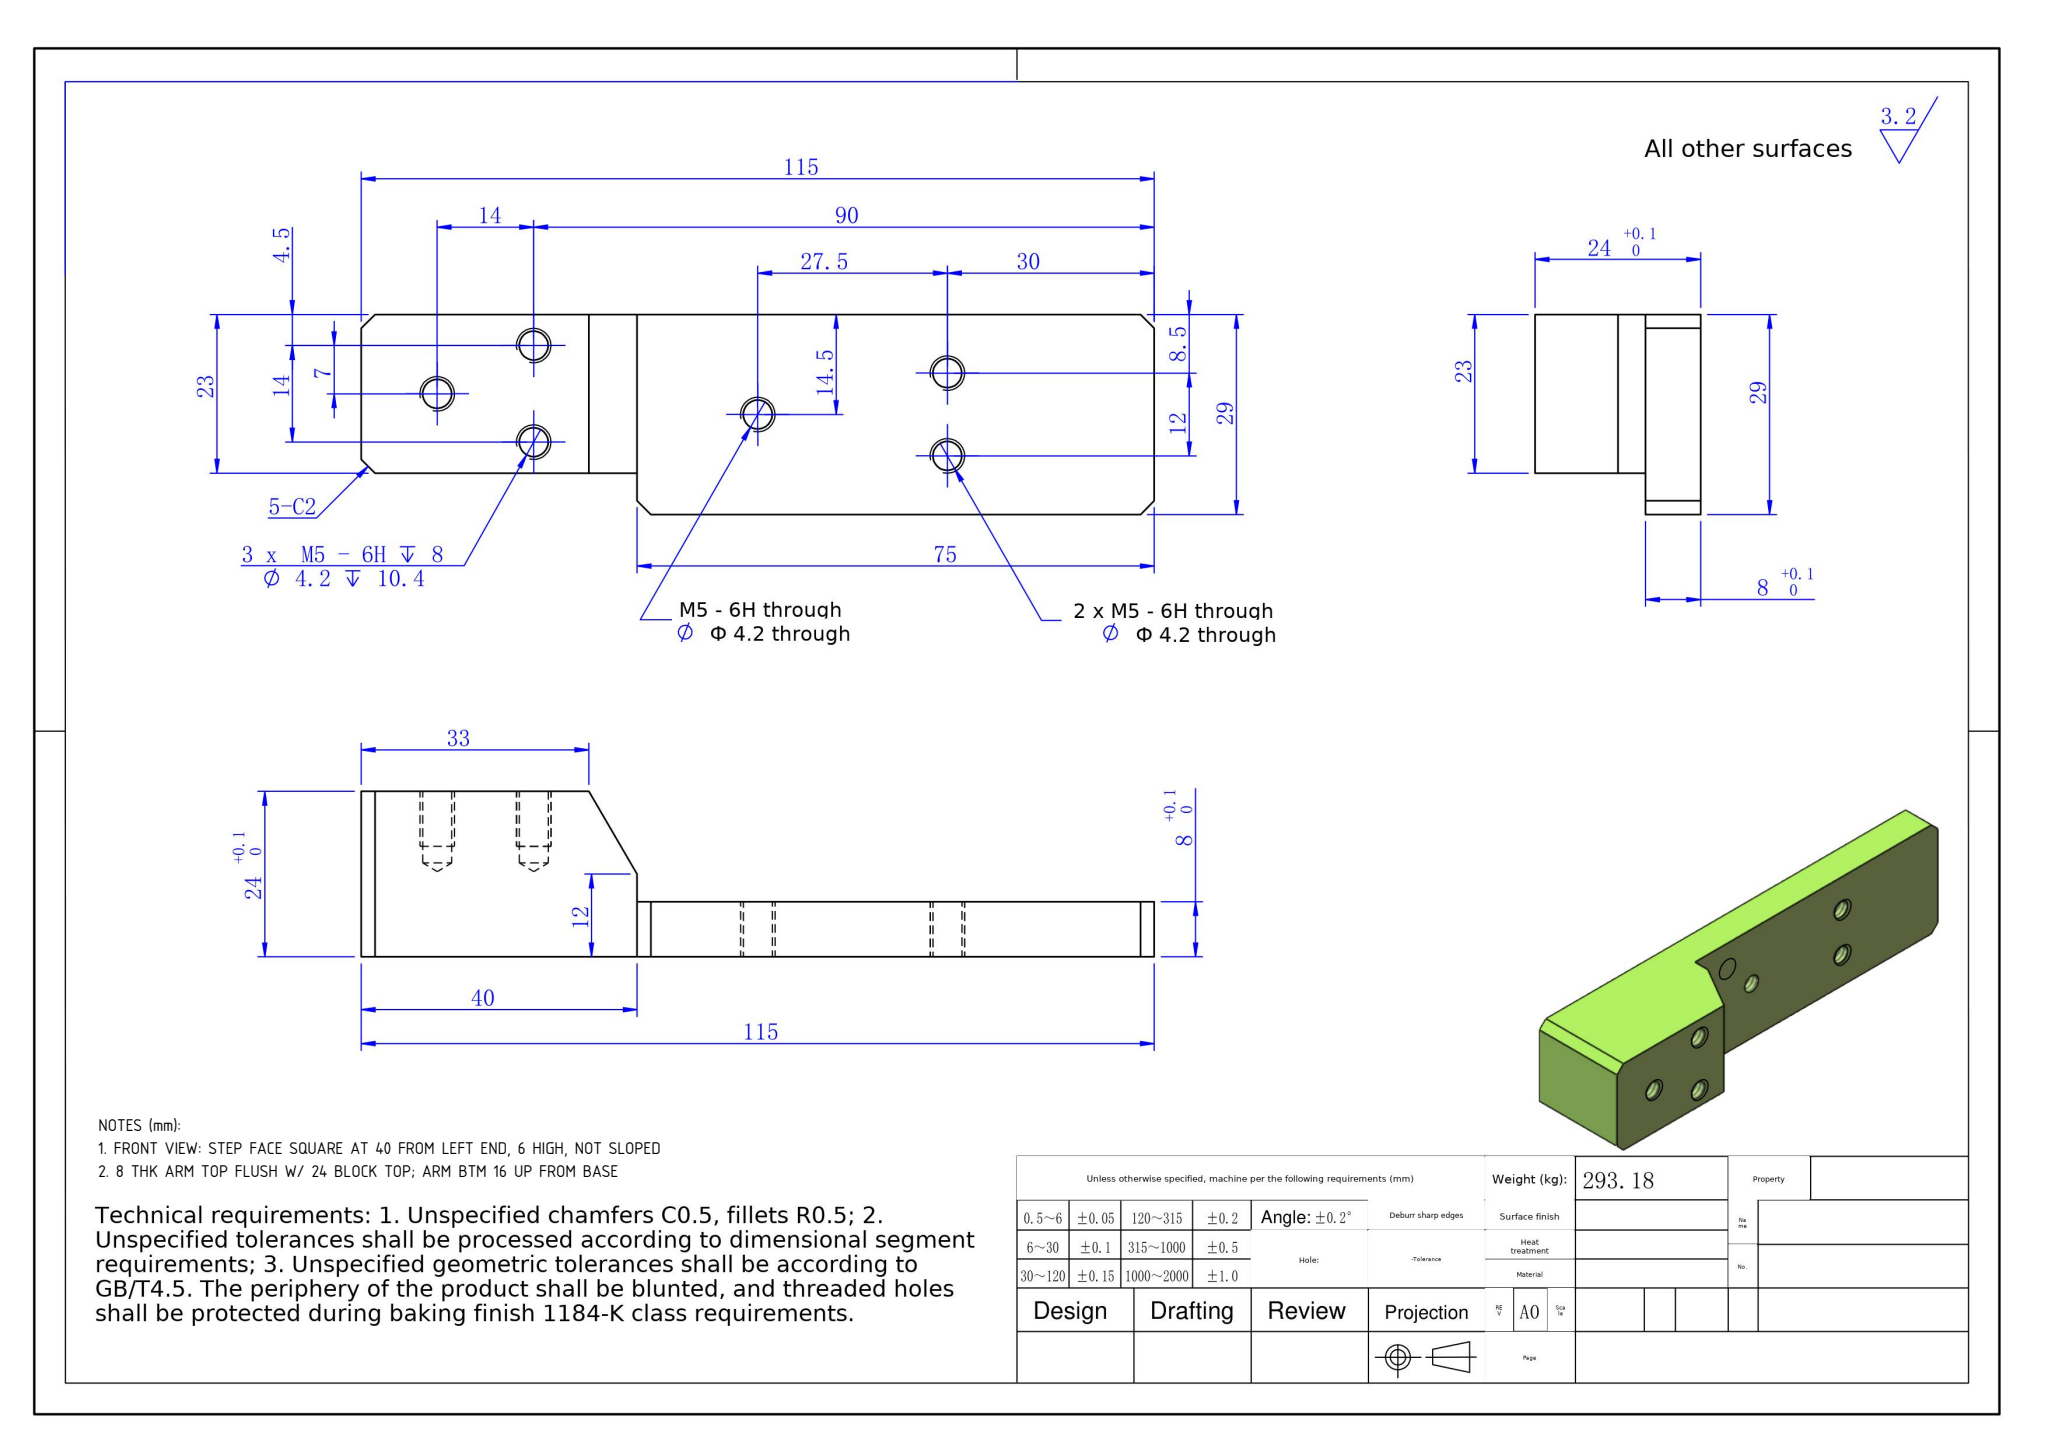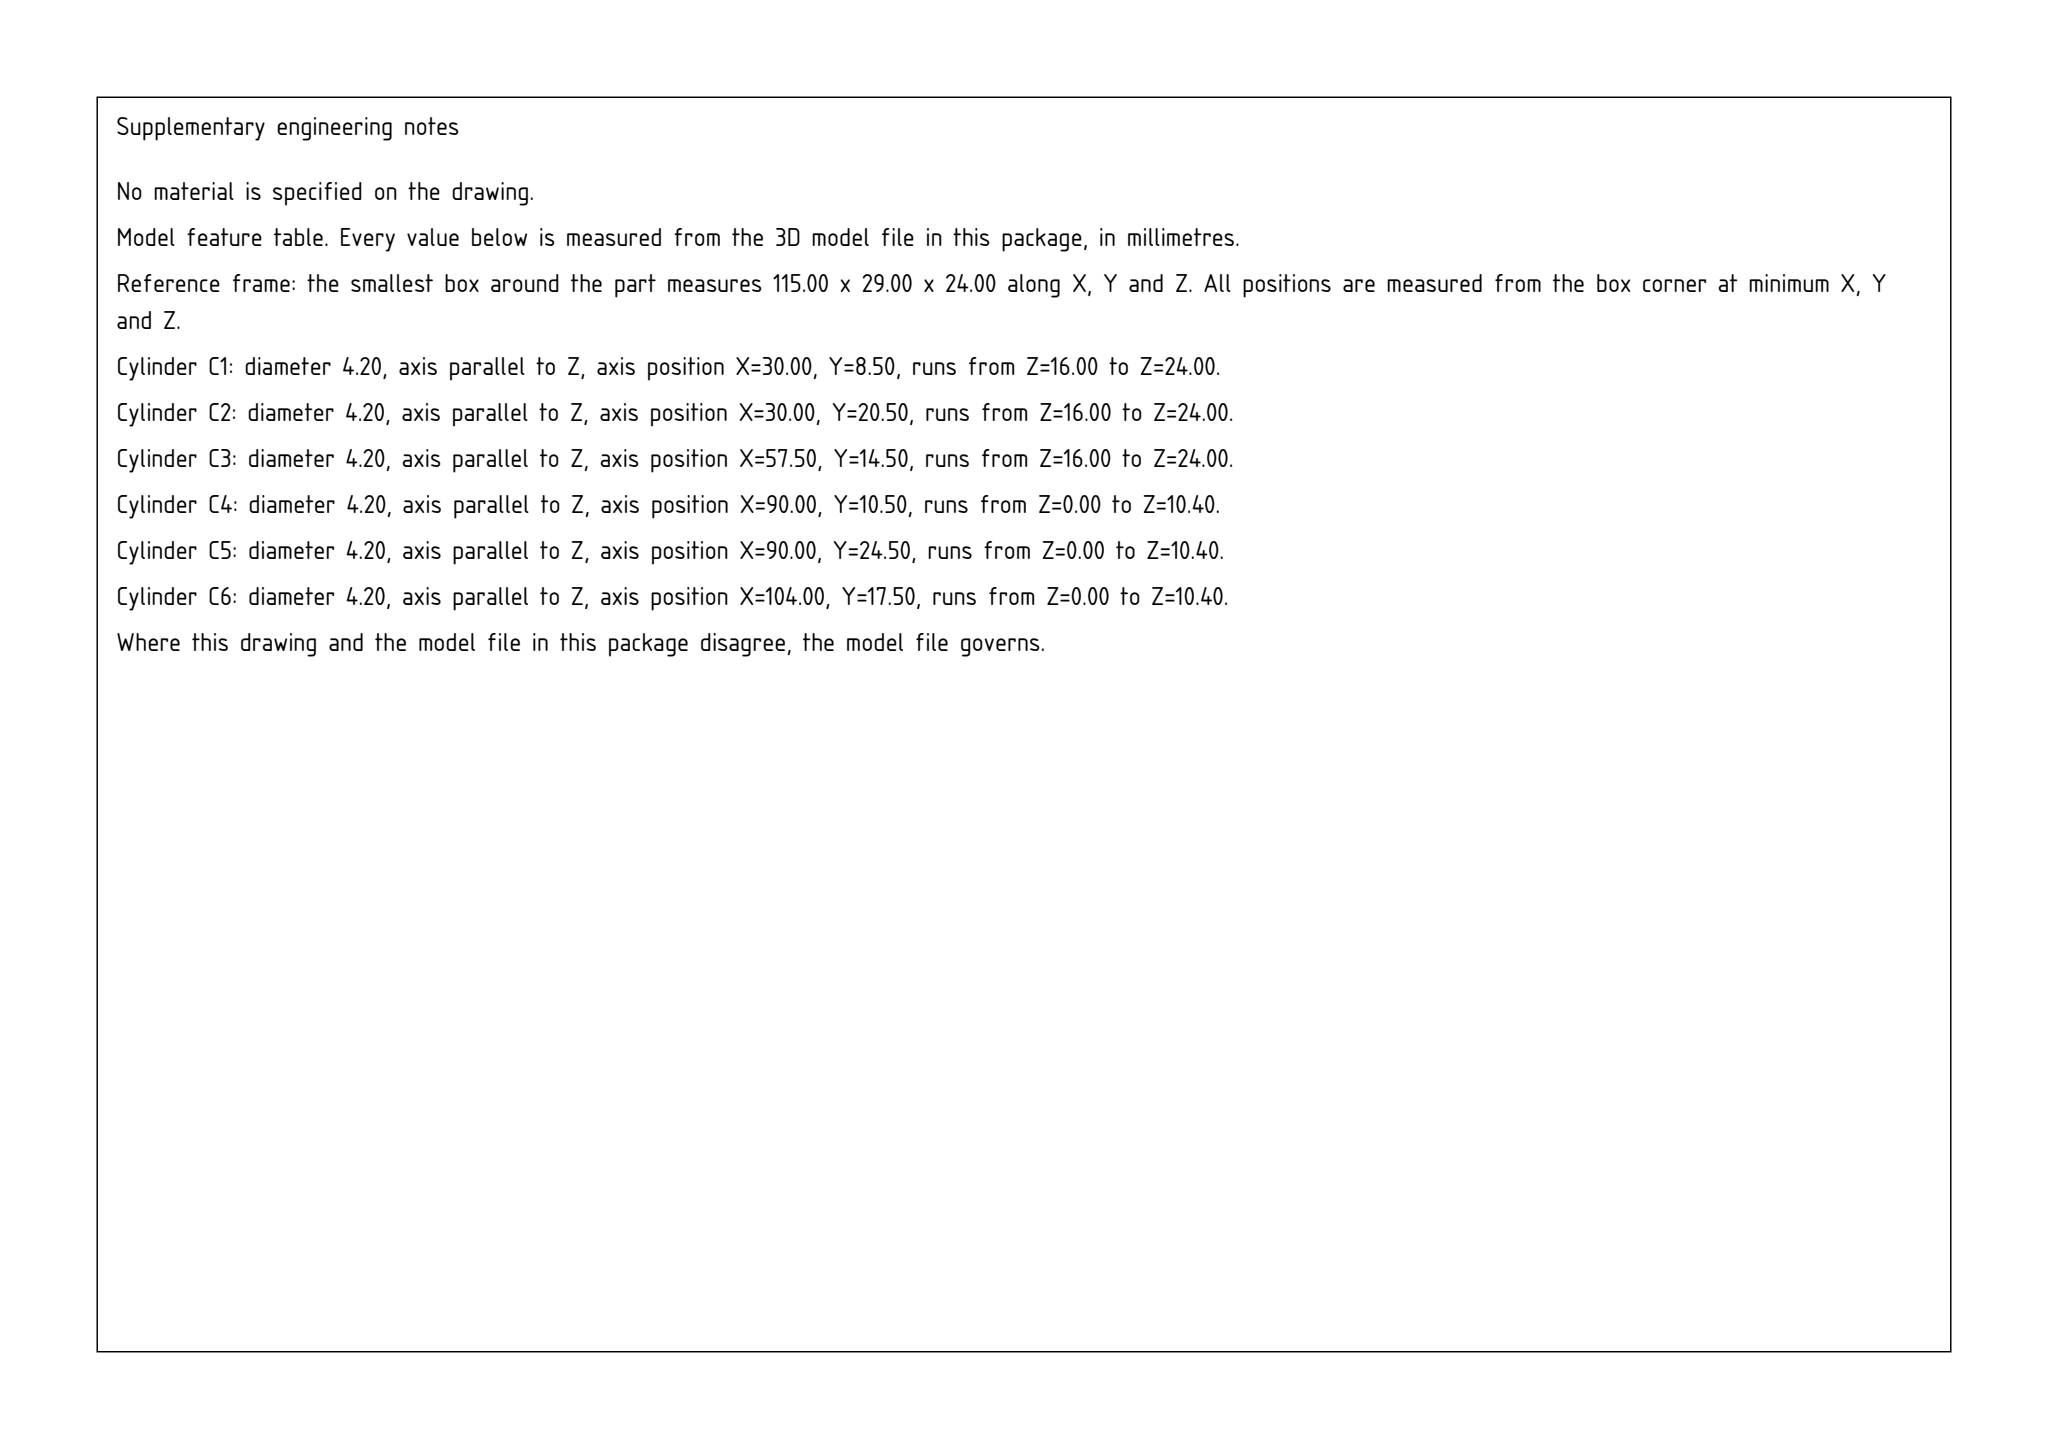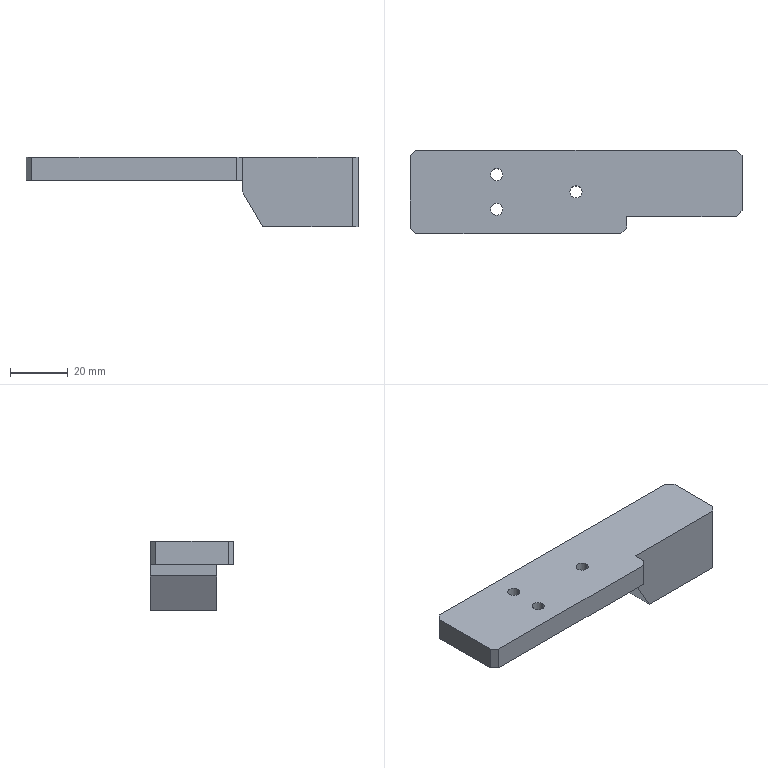Part | SolidWorks | mm | 1 solid | 34 faces | box 115 x 29 x 24 mm | volume 37588 mm3 | plane 16 | cylinder 12 | cone 6 | commonest cylinder face diameters 4.2 x12
Drawing notes:
FRONT VIEW: STEP FACE SQUARE AT 40 FROM LEFT END, 6 HIGH, NOT SLOPED | from the solid: axis_planes x=75.0 count 2 (=115-40 from left end); y-planes 0.0 and 6.0 give 6 step; no non-axis plane at transition
8 THK ARM TOP FLUSH W/ 24 BLOCK TOP; ARM BTM 16 UP FROM BASE | from the solid: z planes at 0, 16, 24; arm thickness 8 spans z16-z24, block spans z0-z24
build123d program:
from build123d import *

# Parameters (mm, degrees)
SKETCH1_W             = 115
SKETCH1_H             = 29
BOSS_EXTRUDE1_DEPTH   = 12
CHAMFER1_SIZE         = 2
M5_TAPPED_HOLE1_D     = 4.2
SKETCH4_W             = 40
SKETCH4_H             = 6
CUT_EXTRUDE1_DEPTH    = 64.973
CHAMFER2_SIZE         = 2
M5_TAPPED_HOLE3_D     = 4.2
M5_TAPPED_HOLE3_DEPTH = 10.4
M5_TAPPED_HOLE3_TIP   = 1.262
M5_TAPPED_HOLE4_D     = 4.2
SKETCH12_W            = 75
SKETCH12_H            = 29
CUT_EXTRUDE3_DEPTH    = 16
CHAMFER3_SIZE         = 7
CHAMFER3_SIZE2        = 12


with BuildPart() as part:
    # Sketch1 → Boss-Extrude1 (new, symmetric)
    with BuildSketch(Plane.XY):
        Rectangle(SKETCH1_W, SKETCH1_H)
    extrude(amount=BOSS_EXTRUDE1_DEPTH, both=True)

    # Chamfer1
    chamfer1_edges = [part.edges().sort_by_distance(p)[0] for p in [
        (57.5, -14.5, 0),
        (-57.5, -14.5, 0),
        (-57.5, 14.5, 0),
        (57.5, 14.5, 0),
    ]]
    chamfer(chamfer1_edges, length=CHAMFER1_SIZE)

    # M5 Tapped Hole1 (through all)
    with Locations(Plane(origin=(0, 0, -12), x_dir=(-1, 0, 0), z_dir=(0, 0, -1))):
        with Locations((27.5, -6), (27.5, 6)):
            Hole(M5_TAPPED_HOLE1_D / 2)

    # Sketch4 → Cut-Extrude1 (cut, through all)
    with BuildSketch(Plane.XY.offset(12)):
        with Locations((37.5, -11.5)):
            Rectangle(SKETCH4_W, SKETCH4_H)
    extrude(amount=-CUT_EXTRUDE1_DEPTH, mode=Mode.SUBTRACT)

    # Chamfer2
    chamfer2_edges = [part.edges().sort_by_distance(p)[0] for p in [
        (57.5, -8.5, 0),
        (17.5, -14.5, 0),
    ]]
    chamfer(chamfer2_edges, length=CHAMFER2_SIZE)

    # M5 Tapped Hole3
    with Locations(Plane(origin=(0, 0, -12), x_dir=(-1, 0, 0), z_dir=(0, 0, -1))):
        with Locations((-32.5, 10), (-32.5, -4), (-46.5, 3)):
            Hole(M5_TAPPED_HOLE3_D / 2, depth=M5_TAPPED_HOLE3_DEPTH)
            with Locations((0, 0, -(M5_TAPPED_HOLE3_DEPTH + M5_TAPPED_HOLE3_TIP / 2))):  # 118° drill point
                Cone(0, M5_TAPPED_HOLE3_D / 2, M5_TAPPED_HOLE3_TIP, mode=Mode.SUBTRACT)

    # M5 Tapped Hole4 (through all)
    with Locations(Plane.XY.offset(12)):
        with Locations((0, 0)):
            Hole(M5_TAPPED_HOLE4_D / 2)

    # Sketch12 → Cut-Extrude3 (cut)
    with BuildSketch(Plane(origin=(0, 0, -12), x_dir=(-1, 0, 0), z_dir=(0, 0, -1))):
        with Locations((20, 0)):
            Rectangle(SKETCH12_W, SKETCH12_H)
    extrude(amount=-CUT_EXTRUDE3_DEPTH, mode=Mode.SUBTRACT)

    # Chamfer3
    chamfer3_edges = [part.edges().sort_by_distance(p)[0] for p in [
        (17.5, 3, -12),
    ]]
    chamfer3_side = [part.faces().sort_by_distance(p)[0] for p in [
        (37.427, 3, -12),
    ]]
    chamfer(chamfer3_edges, length=CHAMFER3_SIZE, length2=CHAMFER3_SIZE2, reference=chamfer3_side[0])


solid = part.part